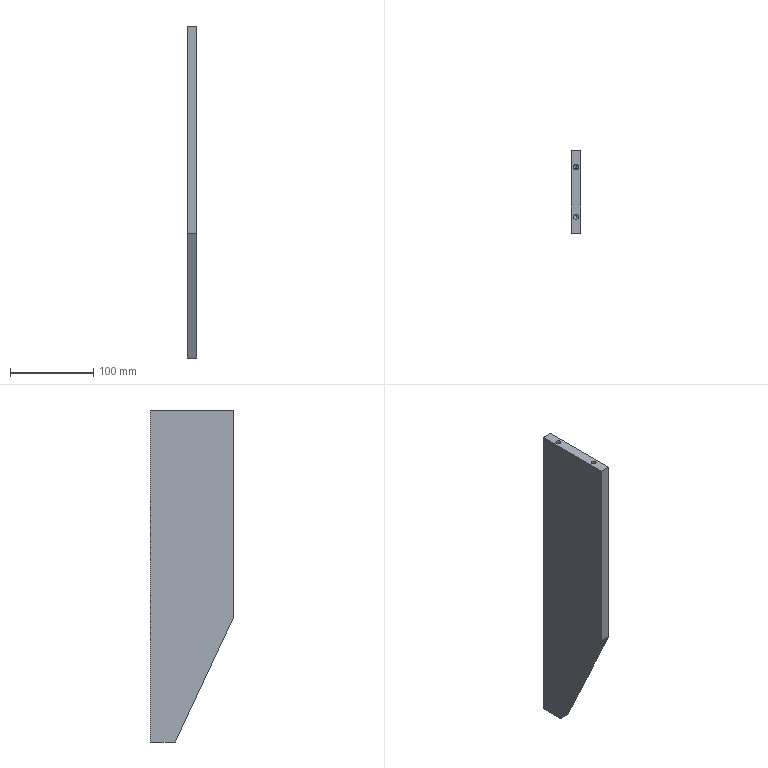Component | SolidWorks | 8TC-A15004-80-03A-1 | 1 solid | 31 faces | box 12 x 100 x 400 mm | volume 414014 mm3 | cylinder 12 | cone 12 | plane 7 | commonest cylinder face diameters 6 x12 | material A3
build123d program:
from build123d import *

# Parameters (mm, degrees)
BOSS_EXTRUDE1_DEPTH   = 6
M6_TAPPED_HOLE1_D     = 6
M6_TAPPED_HOLE1_DEPTH = 17
M6_TAPPED_HOLE1_TIP   = 1.803
M6_TAPPED_HOLE2_D     = 6
M6_TAPPED_HOLE2_DEPTH = 17
M6_TAPPED_HOLE2_TIP   = 1.803


with BuildPart() as part:
    # Sketch1 → Boss-Extrude1 (new, symmetric)
    with BuildSketch(Plane(origin=(0, 0, 0), x_dir=(1, 0, 0), z_dir=(0, 1, 0))):
        Polygon((0, 0), (0, 400), (30, 400), (100, 250), (100, 0), align=None)
    extrude(amount=BOSS_EXTRUDE1_DEPTH, both=True)

    # M6 Tapped Hole1
    with Locations(Plane.XY):
        with Locations((20, 0), (80, 0)):
            Hole(M6_TAPPED_HOLE1_D / 2, depth=M6_TAPPED_HOLE1_DEPTH)
            with Locations((0, 0, -(M6_TAPPED_HOLE1_DEPTH + M6_TAPPED_HOLE1_TIP / 2))):  # 118° drill point
                Cone(0, M6_TAPPED_HOLE1_D / 2, M6_TAPPED_HOLE1_TIP, mode=Mode.SUBTRACT)

    # M6 Tapped Hole2
    with Locations(Plane.ZY):
        with Locations((-50, 0), (-150, 0), (-250, 0), (-350, 0)):
            Hole(M6_TAPPED_HOLE2_D / 2, depth=M6_TAPPED_HOLE2_DEPTH)
            with Locations((0, 0, -(M6_TAPPED_HOLE2_DEPTH + M6_TAPPED_HOLE2_TIP / 2))):  # 118° drill point
                Cone(0, M6_TAPPED_HOLE2_D / 2, M6_TAPPED_HOLE2_TIP, mode=Mode.SUBTRACT)


solid = part.part

# Placed as in the assembly
solid = solid.moved(Location((54, -7.5, 0), (0, 0, -90)))
STEP:
#1=COLOUR_RGB('',0.7922,0.8196,0.9333);
#2=FILL_AREA_STYLE_COLOUR('',#1);
#3=FILL_AREA_STYLE('',(#2));
#4=SURFACE_STYLE_FILL_AREA(#3);
#5=SURFACE_SIDE_STYLE('',(#4));
#6=SURFACE_STYLE_USAGE(.BOTH.,#5);
#7=PRESENTATION_STYLE_ASSIGNMENT((#6));
#8=CARTESIAN_POINT('',(2.126,-0.9646,-2.087));
#9=VERTEX_POINT('',#8);
#10=CARTESIAN_POINT('',(2.126,-0.9646,-1.85));
#11=VERTEX_POINT('',#10);
#12=CARTESIAN_POINT('',(2.126,-0.9646,-1.969));
#13=DIRECTION('',(-0.,1.,0.));
#14=DIRECTION('',(0.,0.,1.));
#15=AXIS2_PLACEMENT_3D('',#12,#13,#14);
#16=CIRCLE('',#15,0.1181);
#17=EDGE_CURVE('',#9,#11,#16,.T.);
#18=ORIENTED_EDGE('',*,*,#17,.F.);
#19=CARTESIAN_POINT('',(2.126,-0.2953,-2.087));
#20=VERTEX_POINT('',#19);
#21=CARTESIAN_POINT('',(2.126,-0.2953,-2.087));
#22=DIRECTION('',(-0.,1.,0.));
#23=VECTOR('',#22,39.37);
#24=LINE('',#21,#23);
#25=EDGE_CURVE('',#9,#20,#24,.T.);
#26=ORIENTED_EDGE('',*,*,#25,.T.);
#27=CARTESIAN_POINT('',(2.126,-0.2953,-1.85));
#28=VERTEX_POINT('',#27);
#29=CARTESIAN_POINT('',(2.126,-0.2953,-1.969));
#30=DIRECTION('',(-0.,1.,0.));
#31=DIRECTION('',(0.,0.,1.));
#32=AXIS2_PLACEMENT_3D('',#29,#30,#31);
#33=CIRCLE('',#32,0.1181);
#34=EDGE_CURVE('',#20,#28,#33,.T.);
#35=ORIENTED_EDGE('',*,*,#34,.T.);
#36=CARTESIAN_POINT('',(2.126,-0.2953,-1.85));
#37=DIRECTION('',(-0.,1.,0.));
#38=VECTOR('',#37,39.37);
#39=LINE('',#36,#38);
#40=EDGE_CURVE('',#11,#28,#39,.T.);
#41=ORIENTED_EDGE('',*,*,#40,.F.);
#42=EDGE_LOOP('',(#18,#26,#35,#41));
#43=FACE_OUTER_BOUND('',#42,.T.);
#44=CARTESIAN_POINT('',(2.126,-0.2953,-1.969));
#45=DIRECTION('',(-0.,1.,0.));
#46=DIRECTION('',(0.,0.,1.));
#47=AXIS2_PLACEMENT_3D('',#44,#45,#46);
#48=CYLINDRICAL_SURFACE('',#47,0.1181);
#49=ADVANCED_FACE('',(#43),#48,.F.);
#50=CARTESIAN_POINT('',(2.126,-1.036,-1.969));
#51=VERTEX_POINT('',#50);
#52=CARTESIAN_POINT('',(2.126,-0.9646,-1.85));
#53=DIRECTION('',(-0.,0.515,0.8572));
#54=VECTOR('',#53,39.37);
#55=LINE('',#52,#54);
#56=EDGE_CURVE('',#51,#11,#55,.T.);
#57=ORIENTED_EDGE('',*,*,#56,.F.);
#58=CARTESIAN_POINT('',(2.126,-0.9646,-2.087));
#59=DIRECTION('',(0.,0.515,-0.8572));
#60=VECTOR('',#59,39.37);
#61=LINE('',#58,#60);
#62=EDGE_CURVE('',#51,#9,#61,.T.);
#63=ORIENTED_EDGE('',*,*,#62,.T.);
#64=ORIENTED_EDGE('',*,*,#17,.T.);
#65=EDGE_LOOP('',(#57,#63,#64));
#66=FACE_OUTER_BOUND('',#65,.T.);
#67=CARTESIAN_POINT('',(2.126,-0.9646,-1.969));
#68=DIRECTION('',(-0.,1.,0.));
#69=DIRECTION('',(0.,0.,1.));
#70=AXIS2_PLACEMENT_3D('',#67,#68,#69);
#71=CONICAL_SURFACE('',#70,0.1181,1.03);
#72=ADVANCED_FACE('',(#66),#71,.F.);
#73=CARTESIAN_POINT('',(2.126,-0.9646,-6.024));
#74=VERTEX_POINT('',#73);
#75=CARTESIAN_POINT('',(2.126,-0.9646,-5.787));
#76=VERTEX_POINT('',#75);
#77=CARTESIAN_POINT('',(2.126,-0.9646,-5.906));
#78=DIRECTION('',(-0.,1.,0.));
#79=DIRECTION('',(0.,0.,1.));
#80=AXIS2_PLACEMENT_3D('',#77,#78,#79);
#81=CIRCLE('',#80,0.1181);
#82=EDGE_CURVE('',#74,#76,#81,.T.);
#83=ORIENTED_EDGE('',*,*,#82,.F.);
#84=CARTESIAN_POINT('',(2.126,-0.2953,-6.024));
#85=VERTEX_POINT('',#84);
#86=CARTESIAN_POINT('',(2.126,-0.2953,-6.024));
#87=DIRECTION('',(-0.,1.,0.));
#88=VECTOR('',#87,39.37);
#89=LINE('',#86,#88);
#90=EDGE_CURVE('',#74,#85,#89,.T.);
#91=ORIENTED_EDGE('',*,*,#90,.T.);
#92=CARTESIAN_POINT('',(2.126,-0.2953,-5.787));
#93=VERTEX_POINT('',#92);
#94=CARTESIAN_POINT('',(2.126,-0.2953,-5.906));
#95=DIRECTION('',(-0.,1.,0.));
#96=DIRECTION('',(0.,0.,1.));
#97=AXIS2_PLACEMENT_3D('',#94,#95,#96);
#98=CIRCLE('',#97,0.1181);
#99=EDGE_CURVE('',#85,#93,#98,.T.);
#100=ORIENTED_EDGE('',*,*,#99,.T.);
#101=CARTESIAN_POINT('',(2.126,-0.2953,-5.787));
#102=DIRECTION('',(-0.,1.,0.));
#103=VECTOR('',#102,39.37);
#104=LINE('',#101,#103);
#105=EDGE_CURVE('',#76,#93,#104,.T.);
#106=ORIENTED_EDGE('',*,*,#105,.F.);
#107=EDGE_LOOP('',(#83,#91,#100,#106));
#108=FACE_OUTER_BOUND('',#107,.T.);
#109=CARTESIAN_POINT('',(2.126,-0.2953,-5.906));
#110=DIRECTION('',(-0.,1.,0.));
#111=DIRECTION('',(0.,0.,1.));
#112=AXIS2_PLACEMENT_3D('',#109,#110,#111);
#113=CYLINDRICAL_SURFACE('',#112,0.1181);
#114=ADVANCED_FACE('',(#108),#113,.F.);
#115=CARTESIAN_POINT('',(2.126,-1.036,-5.906));
#116=VERTEX_POINT('',#115);
#117=CARTESIAN_POINT('',(2.126,-0.9646,-5.787));
#118=DIRECTION('',(-0.,0.515,0.8572));
#119=VECTOR('',#118,39.37);
#120=LINE('',#117,#119);
#121=EDGE_CURVE('',#116,#76,#120,.T.);
#122=ORIENTED_EDGE('',*,*,#121,.F.);
#123=CARTESIAN_POINT('',(2.126,-0.9646,-6.024));
#124=DIRECTION('',(0.,0.515,-0.8572));
#125=VECTOR('',#124,39.37);
#126=LINE('',#123,#125);
#127=EDGE_CURVE('',#116,#74,#126,.T.);
#128=ORIENTED_EDGE('',*,*,#127,.T.);
#129=ORIENTED_EDGE('',*,*,#82,.T.);
#130=EDGE_LOOP('',(#122,#128,#129));
#131=FACE_OUTER_BOUND('',#130,.T.);
#132=CARTESIAN_POINT('',(2.126,-0.9646,-5.906));
#133=DIRECTION('',(-0.,1.,0.));
#134=DIRECTION('',(0.,0.,1.));
#135=AXIS2_PLACEMENT_3D('',#132,#133,#134);
#136=CONICAL_SURFACE('',#135,0.1181,1.03);
#137=ADVANCED_FACE('',(#131),#136,.F.);
#138=CARTESIAN_POINT('',(2.126,-0.9646,-9.961));
#139=VERTEX_POINT('',#138);
#140=CARTESIAN_POINT('',(2.126,-0.9646,-9.724));
#141=VERTEX_POINT('',#140);
#142=CARTESIAN_POINT('',(2.126,-0.9646,-9.843));
#143=DIRECTION('',(-0.,1.,0.));
#144=DIRECTION('',(0.,0.,1.));
#145=AXIS2_PLACEMENT_3D('',#142,#143,#144);
#146=CIRCLE('',#145,0.1181);
#147=EDGE_CURVE('',#139,#141,#146,.T.);
#148=ORIENTED_EDGE('',*,*,#147,.F.);
#149=CARTESIAN_POINT('',(2.126,-0.2953,-9.961));
#150=VERTEX_POINT('',#149);
#151=CARTESIAN_POINT('',(2.126,-0.2953,-9.961));
#152=DIRECTION('',(-0.,1.,0.));
#153=VECTOR('',#152,39.37);
#154=LINE('',#151,#153);
#155=EDGE_CURVE('',#139,#150,#154,.T.);
#156=ORIENTED_EDGE('',*,*,#155,.T.);
#157=CARTESIAN_POINT('',(2.126,-0.2953,-9.724));
#158=VERTEX_POINT('',#157);
#159=CARTESIAN_POINT('',(2.126,-0.2953,-9.843));
#160=DIRECTION('',(-0.,1.,0.));
#161=DIRECTION('',(0.,0.,1.));
#162=AXIS2_PLACEMENT_3D('',#159,#160,#161);
#163=CIRCLE('',#162,0.1181);
#164=EDGE_CURVE('',#150,#158,#163,.T.);
#165=ORIENTED_EDGE('',*,*,#164,.T.);
#166=CARTESIAN_POINT('',(2.126,-0.2953,-9.724));
#167=DIRECTION('',(-0.,1.,0.));
#168=VECTOR('',#167,39.37);
#169=LINE('',#166,#168);
#170=EDGE_CURVE('',#141,#158,#169,.T.);
#171=ORIENTED_EDGE('',*,*,#170,.F.);
#172=EDGE_LOOP('',(#148,#156,#165,#171));
#173=FACE_OUTER_BOUND('',#172,.T.);
#174=CARTESIAN_POINT('',(2.126,-0.2953,-9.843));
#175=DIRECTION('',(-0.,1.,0.));
#176=DIRECTION('',(0.,0.,1.));
#177=AXIS2_PLACEMENT_3D('',#174,#175,#176);
#178=CYLINDRICAL_SURFACE('',#177,0.1181);
#179=ADVANCED_FACE('',(#173),#178,.F.);
#180=CARTESIAN_POINT('',(2.126,-1.036,-9.843));
#181=VERTEX_POINT('',#180);
#182=CARTESIAN_POINT('',(2.126,-0.9646,-9.724));
#183=DIRECTION('',(-0.,0.515,0.8572));
#184=VECTOR('',#183,39.37);
#185=LINE('',#182,#184);
#186=EDGE_CURVE('',#181,#141,#185,.T.);
#187=ORIENTED_EDGE('',*,*,#186,.F.);
#188=CARTESIAN_POINT('',(2.126,-0.9646,-9.961));
#189=DIRECTION('',(0.,0.515,-0.8572));
#190=VECTOR('',#189,39.37);
#191=LINE('',#188,#190);
#192=EDGE_CURVE('',#181,#139,#191,.T.);
#193=ORIENTED_EDGE('',*,*,#192,.T.);
#194=ORIENTED_EDGE('',*,*,#147,.T.);
#195=EDGE_LOOP('',(#187,#193,#194));
#196=FACE_OUTER_BOUND('',#195,.T.);
#197=CARTESIAN_POINT('',(2.126,-0.9646,-9.843));
#198=DIRECTION('',(-0.,1.,0.));
#199=DIRECTION('',(0.,0.,1.));
#200=AXIS2_PLACEMENT_3D('',#197,#198,#199);
#201=CONICAL_SURFACE('',#200,0.1181,1.03);
#202=ADVANCED_FACE('',(#196),#201,.F.);
#203=CARTESIAN_POINT('',(2.126,-0.9646,-13.898));
#204=VERTEX_POINT('',#203);
#205=CARTESIAN_POINT('',(2.126,-0.9646,-13.661));
#206=VERTEX_POINT('',#205);
#207=CARTESIAN_POINT('',(2.126,-0.9646,-13.78));
#208=DIRECTION('',(-0.,1.,0.));
#209=DIRECTION('',(0.,0.,1.));
#210=AXIS2_PLACEMENT_3D('',#207,#208,#209);
#211=CIRCLE('',#210,0.1181);
#212=EDGE_CURVE('',#204,#206,#211,.T.);
#213=ORIENTED_EDGE('',*,*,#212,.F.);
#214=CARTESIAN_POINT('',(2.126,-0.2953,-13.898));
#215=VERTEX_POINT('',#214);
#216=CARTESIAN_POINT('',(2.126,-0.2953,-13.898));
#217=DIRECTION('',(-0.,1.,0.));
#218=VECTOR('',#217,39.37);
#219=LINE('',#216,#218);
#220=EDGE_CURVE('',#204,#215,#219,.T.);
#221=ORIENTED_EDGE('',*,*,#220,.T.);
#222=CARTESIAN_POINT('',(2.126,-0.2953,-13.661));
#223=VERTEX_POINT('',#222);
#224=CARTESIAN_POINT('',(2.126,-0.2953,-13.78));
#225=DIRECTION('',(-0.,1.,0.));
#226=DIRECTION('',(0.,0.,1.));
#227=AXIS2_PLACEMENT_3D('',#224,#225,#226);
#228=CIRCLE('',#227,0.1181);
#229=EDGE_CURVE('',#215,#223,#228,.T.);
#230=ORIENTED_EDGE('',*,*,#229,.T.);
#231=CARTESIAN_POINT('',(2.126,-0.2953,-13.661));
#232=DIRECTION('',(-0.,1.,0.));
#233=VECTOR('',#232,39.37);
#234=LINE('',#231,#233);
#235=EDGE_CURVE('',#206,#223,#234,.T.);
#236=ORIENTED_EDGE('',*,*,#235,.F.);
#237=EDGE_LOOP('',(#213,#221,#230,#236));
#238=FACE_OUTER_BOUND('',#237,.T.);
#239=CARTESIAN_POINT('',(2.126,-0.2953,-13.78));
#240=DIRECTION('',(-0.,1.,0.));
#241=DIRECTION('',(0.,0.,1.));
#242=AXIS2_PLACEMENT_3D('',#239,#240,#241);
#243=CYLINDRICAL_SURFACE('',#242,0.1181);
#244=ADVANCED_FACE('',(#238),#243,.F.);
#245=CARTESIAN_POINT('',(2.126,-1.036,-13.78));
#246=VERTEX_POINT('',#245);
#247=CARTESIAN_POINT('',(2.126,-0.9646,-13.661));
#248=DIRECTION('',(-0.,0.515,0.8572));
#249=VECTOR('',#248,39.37);
#250=LINE('',#247,#249);
#251=EDGE_CURVE('',#246,#206,#250,.T.);
#252=ORIENTED_EDGE('',*,*,#251,.F.);
#253=CARTESIAN_POINT('',(2.126,-0.9646,-13.898));
#254=DIRECTION('',(0.,0.515,-0.8572));
#255=VECTOR('',#254,39.37);
#256=LINE('',#253,#255);
#257=EDGE_CURVE('',#246,#204,#256,.T.);
#258=ORIENTED_EDGE('',*,*,#257,.T.);
#259=ORIENTED_EDGE('',*,*,#212,.T.);
#260=EDGE_LOOP('',(#252,#258,#259));
#261=FACE_OUTER_BOUND('',#260,.T.);
#262=CARTESIAN_POINT('',(2.126,-0.9646,-13.78));
#263=DIRECTION('',(-0.,1.,0.));
#264=DIRECTION('',(0.,0.,1.));
#265=AXIS2_PLACEMENT_3D('',#262,#263,#264);
#266=CONICAL_SURFACE('',#265,0.1181,1.03);
#267=ADVANCED_FACE('',(#261),#266,.F.);
#268=CARTESIAN_POINT('',(2.126,-0.9646,-0.6693));
#269=VERTEX_POINT('',#268);
#270=CARTESIAN_POINT('',(2.126,-1.201,-0.6693));
#271=VERTEX_POINT('',#270);
#272=CARTESIAN_POINT('',(2.126,-1.083,-0.6693));
#273=DIRECTION('',(-0.,-0.,1.));
#274=DIRECTION('',(0.,-1.,0.));
#275=AXIS2_PLACEMENT_3D('',#272,#273,#274);
#276=CIRCLE('',#275,0.1181);
#277=EDGE_CURVE('',#269,#271,#276,.T.);
#278=ORIENTED_EDGE('',*,*,#277,.F.);
#279=CARTESIAN_POINT('',(2.126,-0.9646,-0.));
#280=VERTEX_POINT('',#279);
#281=CARTESIAN_POINT('',(2.126,-0.9646,-0.));
#282=DIRECTION('',(-0.,-0.,1.));
#283=VECTOR('',#282,39.37);
#284=LINE('',#281,#283);
#285=EDGE_CURVE('',#269,#280,#284,.T.);
#286=ORIENTED_EDGE('',*,*,#285,.T.);
#287=CARTESIAN_POINT('',(2.126,-1.201,-0.));
#288=VERTEX_POINT('',#287);
#289=CARTESIAN_POINT('',(2.126,-1.083,-0.));
#290=DIRECTION('',(-0.,-0.,1.));
#291=DIRECTION('',(0.,-1.,0.));
#292=AXIS2_PLACEMENT_3D('',#289,#290,#291);
#293=CIRCLE('',#292,0.1181);
#294=EDGE_CURVE('',#280,#288,#293,.T.);
#295=ORIENTED_EDGE('',*,*,#294,.T.);
#296=CARTESIAN_POINT('',(2.126,-1.201,-0.));
#297=DIRECTION('',(-0.,-0.,1.));
#298=VECTOR('',#297,39.37);
#299=LINE('',#296,#298);
#300=EDGE_CURVE('',#271,#288,#299,.T.);
#301=ORIENTED_EDGE('',*,*,#300,.F.);
#302=EDGE_LOOP('',(#278,#286,#295,#301));
#303=FACE_OUTER_BOUND('',#302,.T.);
#304=CARTESIAN_POINT('',(2.126,-1.083,-0.));
#305=DIRECTION('',(-0.,-0.,1.));
#306=DIRECTION('',(0.,-1.,0.));
#307=AXIS2_PLACEMENT_3D('',#304,#305,#306);
#308=CYLINDRICAL_SURFACE('',#307,0.1181);
#309=ADVANCED_FACE('',(#303),#308,.F.);
#310=CARTESIAN_POINT('',(2.126,-1.083,-0.7403));
#311=VERTEX_POINT('',#310);
#312=CARTESIAN_POINT('',(2.126,-1.201,-0.6693));
#313=DIRECTION('',(0.,-0.8572,0.515));
#314=VECTOR('',#313,39.37);
#315=LINE('',#312,#314);
#316=EDGE_CURVE('',#311,#271,#315,.T.);
#317=ORIENTED_EDGE('',*,*,#316,.F.);
#318=CARTESIAN_POINT('',(2.126,-0.9646,-0.6693));
#319=DIRECTION('',(-0.,0.8572,0.515));
#320=VECTOR('',#319,39.37);
#321=LINE('',#318,#320);
#322=EDGE_CURVE('',#311,#269,#321,.T.);
#323=ORIENTED_EDGE('',*,*,#322,.T.);
#324=ORIENTED_EDGE('',*,*,#277,.T.);
#325=EDGE_LOOP('',(#317,#323,#324));
#326=FACE_OUTER_BOUND('',#325,.T.);
#327=CARTESIAN_POINT('',(2.126,-1.083,-0.6693));
#328=DIRECTION('',(-0.,-0.,1.));
#329=DIRECTION('',(0.,-1.,0.));
#330=AXIS2_PLACEMENT_3D('',#327,#328,#329);
#331=CONICAL_SURFACE('',#330,0.1181,1.03);
#332=ADVANCED_FACE('',(#326),#331,.F.);
#333=CARTESIAN_POINT('',(2.126,-3.327,-0.6693));
#334=VERTEX_POINT('',#333);
#335=CARTESIAN_POINT('',(2.126,-3.563,-0.6693));
#336=VERTEX_POINT('',#335);
#337=CARTESIAN_POINT('',(2.126,-3.445,-0.6693));
#338=DIRECTION('',(-0.,-0.,1.));
#339=DIRECTION('',(0.,-1.,0.));
#340=AXIS2_PLACEMENT_3D('',#337,#338,#339);
#341=CIRCLE('',#340,0.1181);
#342=EDGE_CURVE('',#334,#336,#341,.T.);
#343=ORIENTED_EDGE('',*,*,#342,.F.);
#344=CARTESIAN_POINT('',(2.126,-3.327,-0.));
#345=VERTEX_POINT('',#344);
#346=CARTESIAN_POINT('',(2.126,-3.327,-0.));
#347=DIRECTION('',(-0.,-0.,1.));
#348=VECTOR('',#347,39.37);
#349=LINE('',#346,#348);
#350=EDGE_CURVE('',#334,#345,#349,.T.);
#351=ORIENTED_EDGE('',*,*,#350,.T.);
#352=CARTESIAN_POINT('',(2.126,-3.563,-0.));
#353=VERTEX_POINT('',#352);
#354=CARTESIAN_POINT('',(2.126,-3.445,-0.));
#355=DIRECTION('',(-0.,-0.,1.));
#356=DIRECTION('',(0.,-1.,0.));
#357=AXIS2_PLACEMENT_3D('',#354,#355,#356);
#358=CIRCLE('',#357,0.1181);
#359=EDGE_CURVE('',#345,#353,#358,.T.);
#360=ORIENTED_EDGE('',*,*,#359,.T.);
#361=CARTESIAN_POINT('',(2.126,-3.563,-0.));
#362=DIRECTION('',(-0.,-0.,1.));
#363=VECTOR('',#362,39.37);
#364=LINE('',#361,#363);
#365=EDGE_CURVE('',#336,#353,#364,.T.);
#366=ORIENTED_EDGE('',*,*,#365,.F.);
#367=EDGE_LOOP('',(#343,#351,#360,#366));
#368=FACE_OUTER_BOUND('',#367,.T.);
#369=CARTESIAN_POINT('',(2.126,-3.445,-0.));
#370=DIRECTION('',(-0.,-0.,1.));
#371=DIRECTION('',(0.,-1.,0.));
#372=AXIS2_PLACEMENT_3D('',#369,#370,#371);
#373=CYLINDRICAL_SURFACE('',#372,0.1181);
#374=ADVANCED_FACE('',(#368),#373,.F.);
#375=CARTESIAN_POINT('',(2.126,-3.445,-0.7403));
#376=VERTEX_POINT('',#375);
#377=CARTESIAN_POINT('',(2.126,-3.563,-0.6693));
#378=DIRECTION('',(0.,-0.8572,0.515));
#379=VECTOR('',#378,39.37);
#380=LINE('',#377,#379);
#381=EDGE_CURVE('',#376,#336,#380,.T.);
#382=ORIENTED_EDGE('',*,*,#381,.F.);
#383=CARTESIAN_POINT('',(2.126,-3.327,-0.6693));
#384=DIRECTION('',(-0.,0.8572,0.515));
#385=VECTOR('',#384,39.37);
#386=LINE('',#383,#385);
#387=EDGE_CURVE('',#376,#334,#386,.T.);
#388=ORIENTED_EDGE('',*,*,#387,.T.);
#389=ORIENTED_EDGE('',*,*,#342,.T.);
#390=EDGE_LOOP('',(#382,#388,#389));
#391=FACE_OUTER_BOUND('',#390,.T.);
#392=CARTESIAN_POINT('',(2.126,-3.445,-0.6693));
#393=DIRECTION('',(-0.,-0.,1.));
#394=DIRECTION('',(0.,-1.,0.));
#395=AXIS2_PLACEMENT_3D('',#392,#393,#394);
#396=CONICAL_SURFACE('',#395,0.1181,1.03);
#397=ADVANCED_FACE('',(#391),#396,.F.);
#398=CARTESIAN_POINT('',(2.126,-1.083,-0.));
#399=DIRECTION('',(-0.,-0.,1.));
#400=DIRECTION('',(0.,-1.,0.));
#401=AXIS2_PLACEMENT_3D('',#398,#399,#400);
#402=CIRCLE('',#401,0.1181);
#403=EDGE_CURVE('',#288,#280,#402,.T.);
#404=ORIENTED_EDGE('',*,*,#403,.F.);
#405=ORIENTED_EDGE('',*,*,#294,.F.);
#406=EDGE_LOOP('',(#404,#405));
#407=FACE_BOUND('',#406,.T.);
#408=CARTESIAN_POINT('',(2.126,-3.445,-0.));
#409=DIRECTION('',(-0.,-0.,1.));
#410=DIRECTION('',(0.,-1.,0.));
#411=AXIS2_PLACEMENT_3D('',#408,#409,#410);
#412=CIRCLE('',#411,0.1181);
#413=EDGE_CURVE('',#353,#345,#412,.T.);
#414=ORIENTED_EDGE('',*,*,#413,.F.);
#415=ORIENTED_EDGE('',*,*,#359,.F.);
#416=EDGE_LOOP('',(#414,#415));
#417=FACE_BOUND('',#416,.T.);
#418=CARTESIAN_POINT('',(1.89,-0.2953,-0.));
#419=VERTEX_POINT('',#418);
#420=CARTESIAN_POINT('',(1.89,-4.232,-0.));
#421=VERTEX_POINT('',#420);
#422=CARTESIAN_POINT('',(1.89,-4.232,-0.));
#423=DIRECTION('',(0.,-1.,0.));
#424=VECTOR('',#423,39.37);
#425=LINE('',#422,#424);
#426=EDGE_CURVE('',#419,#421,#425,.T.);
#427=ORIENTED_EDGE('',*,*,#426,.T.);
#428=CARTESIAN_POINT('',(2.362,-4.232,-0.));
#429=VERTEX_POINT('',#428);
#430=CARTESIAN_POINT('',(2.362,-4.232,-0.));
#431=DIRECTION('',(-1.,-0.,-0.));
#432=VECTOR('',#431,39.37);
#433=LINE('',#430,#432);
#434=EDGE_CURVE('',#429,#421,#433,.T.);
#435=ORIENTED_EDGE('',*,*,#434,.F.);
#436=CARTESIAN_POINT('',(2.362,-0.2953,-0.));
#437=VERTEX_POINT('',#436);
#438=CARTESIAN_POINT('',(2.362,-4.232,-0.));
#439=DIRECTION('',(0.,-1.,0.));
#440=VECTOR('',#439,39.37);
#441=LINE('',#438,#440);
#442=EDGE_CURVE('',#437,#429,#441,.T.);
#443=ORIENTED_EDGE('',*,*,#442,.F.);
#444=CARTESIAN_POINT('',(2.362,-0.2953,-0.));
#445=DIRECTION('',(-1.,-0.,-0.));
#446=VECTOR('',#445,39.37);
#447=LINE('',#444,#446);
#448=EDGE_CURVE('',#437,#419,#447,.T.);
#449=ORIENTED_EDGE('',*,*,#448,.T.);
#450=EDGE_LOOP('',(#427,#435,#443,#449));
#451=FACE_OUTER_BOUND('',#450,.T.);
#452=CARTESIAN_POINT('',(2.362,-4.232,-0.));
#453=DIRECTION('',(0.,0.,-1.));
#454=DIRECTION('',(-0.,1.,0.));
#455=AXIS2_PLACEMENT_3D('',#452,#453,#454);
#456=PLANE('',#455);
#457=ADVANCED_FACE('',(#407,#417,#451),#456,.F.);
#458=CARTESIAN_POINT('',(1.89,-4.232,-9.843));
#459=VERTEX_POINT('',#458);
#460=CARTESIAN_POINT('',(1.89,-4.232,-9.843));
#461=DIRECTION('',(0.,0.,-1.));
#462=VECTOR('',#461,39.37);
#463=LINE('',#460,#462);
#464=EDGE_CURVE('',#421,#459,#463,.T.);
#465=ORIENTED_EDGE('',*,*,#464,.T.);
#466=CARTESIAN_POINT('',(2.362,-4.232,-9.843));
#467=VERTEX_POINT('',#466);
#468=CARTESIAN_POINT('',(2.362,-4.232,-9.843));
#469=DIRECTION('',(-1.,-0.,-0.));
#470=VECTOR('',#469,39.37);
#471=LINE('',#468,#470);
#472=EDGE_CURVE('',#467,#459,#471,.T.);
#473=ORIENTED_EDGE('',*,*,#472,.F.);
#474=CARTESIAN_POINT('',(2.362,-4.232,-9.843));
#475=DIRECTION('',(0.,0.,-1.));
#476=VECTOR('',#475,39.37);
#477=LINE('',#474,#476);
#478=EDGE_CURVE('',#429,#467,#477,.T.);
#479=ORIENTED_EDGE('',*,*,#478,.F.);
#480=ORIENTED_EDGE('',*,*,#434,.T.);
#481=EDGE_LOOP('',(#465,#473,#479,#480));
#482=FACE_OUTER_BOUND('',#481,.T.);
#483=CARTESIAN_POINT('',(2.362,-4.232,-9.843));
#484=DIRECTION('',(-0.,1.,0.));
#485=DIRECTION('',(-0.,-0.,1.));
#486=AXIS2_PLACEMENT_3D('',#483,#484,#485);
#487=PLANE('',#486);
#488=ADVANCED_FACE('',(#482),#487,.F.);
#489=CARTESIAN_POINT('',(1.89,-1.476,-15.748));
#490=VERTEX_POINT('',#489);
#491=CARTESIAN_POINT('',(1.89,-1.476,-15.748));
#492=DIRECTION('',(-0.,0.4229,-0.9062));
#493=VECTOR('',#492,39.37);
#494=LINE('',#491,#493);
#495=EDGE_CURVE('',#459,#490,#494,.T.);
#496=ORIENTED_EDGE('',*,*,#495,.T.);
#497=CARTESIAN_POINT('',(2.362,-1.476,-15.748));
#498=VERTEX_POINT('',#497);
#499=CARTESIAN_POINT('',(2.362,-1.476,-15.748));
#500=DIRECTION('',(-1.,-0.,-0.));
#501=VECTOR('',#500,39.37);
#502=LINE('',#499,#501);
#503=EDGE_CURVE('',#498,#490,#502,.T.);
#504=ORIENTED_EDGE('',*,*,#503,.F.);
#505=CARTESIAN_POINT('',(2.362,-1.476,-15.748));
#506=DIRECTION('',(-0.,0.4229,-0.9062));
#507=VECTOR('',#506,39.37);
#508=LINE('',#505,#507);
#509=EDGE_CURVE('',#467,#498,#508,.T.);
#510=ORIENTED_EDGE('',*,*,#509,.F.);
#511=ORIENTED_EDGE('',*,*,#472,.T.);
#512=EDGE_LOOP('',(#496,#504,#510,#511));
#513=FACE_OUTER_BOUND('',#512,.T.);
#514=CARTESIAN_POINT('',(2.362,-1.476,-15.748));
#515=DIRECTION('',(-0.,0.9062,0.4229));
#516=DIRECTION('',(0.,-0.4229,0.9062));
#517=AXIS2_PLACEMENT_3D('',#514,#515,#516);
#518=PLANE('',#517);
#519=ADVANCED_FACE('',(#513),#518,.F.);
#520=CARTESIAN_POINT('',(1.89,-0.2953,-15.748));
#521=VERTEX_POINT('',#520);
#522=CARTESIAN_POINT('',(1.89,-0.2953,-15.748));
#523=DIRECTION('',(-0.,1.,0.));
#524=VECTOR('',#523,39.37);
#525=LINE('',#522,#524);
#526=EDGE_CURVE('',#490,#521,#525,.T.);
#527=ORIENTED_EDGE('',*,*,#526,.T.);
#528=CARTESIAN_POINT('',(2.362,-0.2953,-15.748));
#529=VERTEX_POINT('',#528);
#530=CARTESIAN_POINT('',(2.362,-0.2953,-15.748));
#531=DIRECTION('',(-1.,-0.,-0.));
#532=VECTOR('',#531,39.37);
#533=LINE('',#530,#532);
#534=EDGE_CURVE('',#529,#521,#533,.T.);
#535=ORIENTED_EDGE('',*,*,#534,.F.);
#536=CARTESIAN_POINT('',(2.362,-0.2953,-15.748));
#537=DIRECTION('',(-0.,1.,0.));
#538=VECTOR('',#537,39.37);
#539=LINE('',#536,#538);
#540=EDGE_CURVE('',#498,#529,#539,.T.);
#541=ORIENTED_EDGE('',*,*,#540,.F.);
#542=ORIENTED_EDGE('',*,*,#503,.T.);
#543=EDGE_LOOP('',(#527,#535,#541,#542));
#544=FACE_OUTER_BOUND('',#543,.T.);
#545=CARTESIAN_POINT('',(2.362,-0.2953,-15.748));
#546=DIRECTION('',(-0.,-0.,1.));
#547=DIRECTION('',(0.,-1.,0.));
#548=AXIS2_PLACEMENT_3D('',#545,#546,#547);
#549=PLANE('',#548);
#550=ADVANCED_FACE('',(#544),#549,.F.);
#551=CARTESIAN_POINT('',(2.126,-0.2953,-1.969));
#552=DIRECTION('',(-0.,1.,0.));
#553=DIRECTION('',(0.,0.,1.));
#554=AXIS2_PLACEMENT_3D('',#551,#552,#553);
#555=CIRCLE('',#554,0.1181);
#556=EDGE_CURVE('',#28,#20,#555,.T.);
#557=ORIENTED_EDGE('',*,*,#556,.F.);
#558=ORIENTED_EDGE('',*,*,#34,.F.);
#559=EDGE_LOOP('',(#557,#558));
#560=FACE_BOUND('',#559,.T.);
#561=CARTESIAN_POINT('',(2.126,-0.2953,-5.906));
#562=DIRECTION('',(-0.,1.,0.));
#563=DIRECTION('',(0.,0.,1.));
#564=AXIS2_PLACEMENT_3D('',#561,#562,#563);
#565=CIRCLE('',#564,0.1181);
#566=EDGE_CURVE('',#93,#85,#565,.T.);
#567=ORIENTED_EDGE('',*,*,#566,.F.);
#568=ORIENTED_EDGE('',*,*,#99,.F.);
#569=EDGE_LOOP('',(#567,#568));
#570=FACE_BOUND('',#569,.T.);
#571=CARTESIAN_POINT('',(2.126,-0.2953,-9.843));
#572=DIRECTION('',(-0.,1.,0.));
#573=DIRECTION('',(0.,0.,1.));
#574=AXIS2_PLACEMENT_3D('',#571,#572,#573);
#575=CIRCLE('',#574,0.1181);
#576=EDGE_CURVE('',#158,#150,#575,.T.);
#577=ORIENTED_EDGE('',*,*,#576,.F.);
#578=ORIENTED_EDGE('',*,*,#164,.F.);
#579=EDGE_LOOP('',(#577,#578));
#580=FACE_BOUND('',#579,.T.);
#581=CARTESIAN_POINT('',(2.126,-0.2953,-13.78));
#582=DIRECTION('',(-0.,1.,0.));
#583=DIRECTION('',(0.,0.,1.));
#584=AXIS2_PLACEMENT_3D('',#581,#582,#583);
#585=CIRCLE('',#584,0.1181);
#586=EDGE_CURVE('',#223,#215,#585,.T.);
#587=ORIENTED_EDGE('',*,*,#586,.F.);
#588=ORIENTED_EDGE('',*,*,#229,.F.);
#589=EDGE_LOOP('',(#587,#588));
#590=FACE_BOUND('',#589,.T.);
#591=CARTESIAN_POINT('',(1.89,-0.2953,-0.));
#592=DIRECTION('',(-0.,-0.,1.));
#593=VECTOR('',#592,39.37);
#594=LINE('',#591,#593);
#595=EDGE_CURVE('',#521,#419,#594,.T.);
#596=ORIENTED_EDGE('',*,*,#595,.T.);
#597=ORIENTED_EDGE('',*,*,#448,.F.);
#598=CARTESIAN_POINT('',(2.362,-0.2953,-0.));
#599=DIRECTION('',(-0.,-0.,1.));
#600=VECTOR('',#599,39.37);
#601=LINE('',#598,#600);
#602=EDGE_CURVE('',#529,#437,#601,.T.);
#603=ORIENTED_EDGE('',*,*,#602,.F.);
#604=ORIENTED_EDGE('',*,*,#534,.T.);
#605=EDGE_LOOP('',(#596,#597,#603,#604));
#606=FACE_OUTER_BOUND('',#605,.T.);
#607=CARTESIAN_POINT('',(2.362,-0.2953,-0.));
#608=DIRECTION('',(0.,-1.,0.));
#609=DIRECTION('',(0.,0.,-1.));
#610=AXIS2_PLACEMENT_3D('',#607,#608,#609);
#611=PLANE('',#610);
#612=ADVANCED_FACE('',(#560,#570,#580,#590,#606),#611,.F.);
#613=ORIENTED_EDGE('',*,*,#442,.T.);
#614=ORIENTED_EDGE('',*,*,#478,.T.);
#615=ORIENTED_EDGE('',*,*,#509,.T.);
#616=ORIENTED_EDGE('',*,*,#540,.T.);
#617=ORIENTED_EDGE('',*,*,#602,.T.);
#618=EDGE_LOOP('',(#613,#614,#615,#616,#617));
#619=FACE_OUTER_BOUND('',#618,.T.);
#620=CARTESIAN_POINT('',(2.362,-0.2953,-0.));
#621=DIRECTION('',(-1.,-0.,-0.));
#622=DIRECTION('',(0.,0.,-1.));
#623=AXIS2_PLACEMENT_3D('',#620,#621,#622);
#624=PLANE('',#623);
#625=ADVANCED_FACE('',(#619),#624,.F.);
#626=ORIENTED_EDGE('',*,*,#426,.F.);
#627=ORIENTED_EDGE('',*,*,#595,.F.);
#628=ORIENTED_EDGE('',*,*,#526,.F.);
#629=ORIENTED_EDGE('',*,*,#495,.F.);
#630=ORIENTED_EDGE('',*,*,#464,.F.);
#631=EDGE_LOOP('',(#626,#627,#628,#629,#630));
#632=FACE_OUTER_BOUND('',#631,.T.);
#633=CARTESIAN_POINT('',(1.89,-0.2953,-0.));
#634=DIRECTION('',(-1.,-0.,-0.));
#635=DIRECTION('',(0.,0.,-1.));
#636=AXIS2_PLACEMENT_3D('',#633,#634,#635);
#637=PLANE('',#636);
#638=ADVANCED_FACE('',(#632),#637,.T.);
#639=ORIENTED_EDGE('',*,*,#387,.F.);
#640=ORIENTED_EDGE('',*,*,#381,.T.);
#641=CARTESIAN_POINT('',(2.126,-3.445,-0.6693));
#642=DIRECTION('',(-0.,-0.,1.));
#643=DIRECTION('',(0.,-1.,0.));
#644=AXIS2_PLACEMENT_3D('',#641,#642,#643);
#645=CIRCLE('',#644,0.1181);
#646=EDGE_CURVE('',#336,#334,#645,.T.);
#647=ORIENTED_EDGE('',*,*,#646,.T.);
#648=EDGE_LOOP('',(#639,#640,#647));
#649=FACE_OUTER_BOUND('',#648,.T.);
#650=CARTESIAN_POINT('',(2.126,-3.445,-0.6693));
#651=DIRECTION('',(-0.,-0.,1.));
#652=DIRECTION('',(0.,-1.,0.));
#653=AXIS2_PLACEMENT_3D('',#650,#651,#652);
#654=CONICAL_SURFACE('',#653,0.1181,1.03);
#655=ADVANCED_FACE('',(#649),#654,.F.);
#656=ORIENTED_EDGE('',*,*,#350,.F.);
#657=ORIENTED_EDGE('',*,*,#646,.F.);
#658=ORIENTED_EDGE('',*,*,#365,.T.);
#659=ORIENTED_EDGE('',*,*,#413,.T.);
#660=EDGE_LOOP('',(#656,#657,#658,#659));
#661=FACE_OUTER_BOUND('',#660,.T.);
#662=CARTESIAN_POINT('',(2.126,-3.445,-0.));
#663=DIRECTION('',(-0.,-0.,1.));
#664=DIRECTION('',(0.,-1.,0.));
#665=AXIS2_PLACEMENT_3D('',#662,#663,#664);
#666=CYLINDRICAL_SURFACE('',#665,0.1181);
#667=ADVANCED_FACE('',(#661),#666,.F.);
#668=ORIENTED_EDGE('',*,*,#322,.F.);
#669=ORIENTED_EDGE('',*,*,#316,.T.);
#670=CARTESIAN_POINT('',(2.126,-1.083,-0.6693));
#671=DIRECTION('',(-0.,-0.,1.));
#672=DIRECTION('',(0.,-1.,0.));
#673=AXIS2_PLACEMENT_3D('',#670,#671,#672);
#674=CIRCLE('',#673,0.1181);
#675=EDGE_CURVE('',#271,#269,#674,.T.);
#676=ORIENTED_EDGE('',*,*,#675,.T.);
#677=EDGE_LOOP('',(#668,#669,#676));
#678=FACE_OUTER_BOUND('',#677,.T.);
#679=CARTESIAN_POINT('',(2.126,-1.083,-0.6693));
#680=DIRECTION('',(-0.,-0.,1.));
#681=DIRECTION('',(0.,-1.,0.));
#682=AXIS2_PLACEMENT_3D('',#679,#680,#681);
#683=CONICAL_SURFACE('',#682,0.1181,1.03);
#684=ADVANCED_FACE('',(#678),#683,.F.);
#685=ORIENTED_EDGE('',*,*,#285,.F.);
#686=ORIENTED_EDGE('',*,*,#675,.F.);
#687=ORIENTED_EDGE('',*,*,#300,.T.);
#688=ORIENTED_EDGE('',*,*,#403,.T.);
#689=EDGE_LOOP('',(#685,#686,#687,#688));
#690=FACE_OUTER_BOUND('',#689,.T.);
#691=CARTESIAN_POINT('',(2.126,-1.083,-0.));
#692=DIRECTION('',(-0.,-0.,1.));
#693=DIRECTION('',(0.,-1.,0.));
#694=AXIS2_PLACEMENT_3D('',#691,#692,#693);
#695=CYLINDRICAL_SURFACE('',#694,0.1181);
#696=ADVANCED_FACE('',(#690),#695,.F.);
#697=ORIENTED_EDGE('',*,*,#257,.F.);
#698=ORIENTED_EDGE('',*,*,#251,.T.);
#699=CARTESIAN_POINT('',(2.126,-0.9646,-13.78));
#700=DIRECTION('',(-0.,1.,0.));
#701=DIRECTION('',(0.,0.,1.));
#702=AXIS2_PLACEMENT_3D('',#699,#700,#701);
#703=CIRCLE('',#702,0.1181);
#704=EDGE_CURVE('',#206,#204,#703,.T.);
#705=ORIENTED_EDGE('',*,*,#704,.T.);
#706=EDGE_LOOP('',(#697,#698,#705));
#707=FACE_OUTER_BOUND('',#706,.T.);
#708=CARTESIAN_POINT('',(2.126,-0.9646,-13.78));
#709=DIRECTION('',(-0.,1.,0.));
#710=DIRECTION('',(0.,0.,1.));
#711=AXIS2_PLACEMENT_3D('',#708,#709,#710);
#712=CONICAL_SURFACE('',#711,0.1181,1.03);
#713=ADVANCED_FACE('',(#707),#712,.F.);
#714=ORIENTED_EDGE('',*,*,#220,.F.);
#715=ORIENTED_EDGE('',*,*,#704,.F.);
#716=ORIENTED_EDGE('',*,*,#235,.T.);
#717=ORIENTED_EDGE('',*,*,#586,.T.);
#718=EDGE_LOOP('',(#714,#715,#716,#717));
#719=FACE_OUTER_BOUND('',#718,.T.);
#720=CARTESIAN_POINT('',(2.126,-0.2953,-13.78));
#721=DIRECTION('',(-0.,1.,0.));
#722=DIRECTION('',(0.,0.,1.));
#723=AXIS2_PLACEMENT_3D('',#720,#721,#722);
#724=CYLINDRICAL_SURFACE('',#723,0.1181);
#725=ADVANCED_FACE('',(#719),#724,.F.);
#726=ORIENTED_EDGE('',*,*,#192,.F.);
#727=ORIENTED_EDGE('',*,*,#186,.T.);
#728=CARTESIAN_POINT('',(2.126,-0.9646,-9.843));
#729=DIRECTION('',(-0.,1.,0.));
#730=DIRECTION('',(0.,0.,1.));
#731=AXIS2_PLACEMENT_3D('',#728,#729,#730);
#732=CIRCLE('',#731,0.1181);
#733=EDGE_CURVE('',#141,#139,#732,.T.);
#734=ORIENTED_EDGE('',*,*,#733,.T.);
#735=EDGE_LOOP('',(#726,#727,#734));
#736=FACE_OUTER_BOUND('',#735,.T.);
#737=CARTESIAN_POINT('',(2.126,-0.9646,-9.843));
#738=DIRECTION('',(-0.,1.,0.));
#739=DIRECTION('',(0.,0.,1.));
#740=AXIS2_PLACEMENT_3D('',#737,#738,#739);
#741=CONICAL_SURFACE('',#740,0.1181,1.03);
#742=ADVANCED_FACE('',(#736),#741,.F.);
#743=ORIENTED_EDGE('',*,*,#155,.F.);
#744=ORIENTED_EDGE('',*,*,#733,.F.);
#745=ORIENTED_EDGE('',*,*,#170,.T.);
#746=ORIENTED_EDGE('',*,*,#576,.T.);
#747=EDGE_LOOP('',(#743,#744,#745,#746));
#748=FACE_OUTER_BOUND('',#747,.T.);
#749=CARTESIAN_POINT('',(2.126,-0.2953,-9.843));
#750=DIRECTION('',(-0.,1.,0.));
#751=DIRECTION('',(0.,0.,1.));
#752=AXIS2_PLACEMENT_3D('',#749,#750,#751);
#753=CYLINDRICAL_SURFACE('',#752,0.1181);
#754=ADVANCED_FACE('',(#748),#753,.F.);
#755=ORIENTED_EDGE('',*,*,#127,.F.);
#756=ORIENTED_EDGE('',*,*,#121,.T.);
#757=CARTESIAN_POINT('',(2.126,-0.9646,-5.906));
#758=DIRECTION('',(-0.,1.,0.));
#759=DIRECTION('',(0.,0.,1.));
#760=AXIS2_PLACEMENT_3D('',#757,#758,#759);
#761=CIRCLE('',#760,0.1181);
#762=EDGE_CURVE('',#76,#74,#761,.T.);
#763=ORIENTED_EDGE('',*,*,#762,.T.);
#764=EDGE_LOOP('',(#755,#756,#763));
#765=FACE_OUTER_BOUND('',#764,.T.);
#766=CARTESIAN_POINT('',(2.126,-0.9646,-5.906));
#767=DIRECTION('',(-0.,1.,0.));
#768=DIRECTION('',(0.,0.,1.));
#769=AXIS2_PLACEMENT_3D('',#766,#767,#768);
#770=CONICAL_SURFACE('',#769,0.1181,1.03);
#771=ADVANCED_FACE('',(#765),#770,.F.);
#772=ORIENTED_EDGE('',*,*,#90,.F.);
#773=ORIENTED_EDGE('',*,*,#762,.F.);
#774=ORIENTED_EDGE('',*,*,#105,.T.);
#775=ORIENTED_EDGE('',*,*,#566,.T.);
#776=EDGE_LOOP('',(#772,#773,#774,#775));
#777=FACE_OUTER_BOUND('',#776,.T.);
#778=CARTESIAN_POINT('',(2.126,-0.2953,-5.906));
#779=DIRECTION('',(-0.,1.,0.));
#780=DIRECTION('',(0.,0.,1.));
#781=AXIS2_PLACEMENT_3D('',#778,#779,#780);
#782=CYLINDRICAL_SURFACE('',#781,0.1181);
#783=ADVANCED_FACE('',(#777),#782,.F.);
#784=ORIENTED_EDGE('',*,*,#62,.F.);
#785=ORIENTED_EDGE('',*,*,#56,.T.);
#786=CARTESIAN_POINT('',(2.126,-0.9646,-1.969));
#787=DIRECTION('',(-0.,1.,0.));
#788=DIRECTION('',(0.,0.,1.));
#789=AXIS2_PLACEMENT_3D('',#786,#787,#788);
#790=CIRCLE('',#789,0.1181);
#791=EDGE_CURVE('',#11,#9,#790,.T.);
#792=ORIENTED_EDGE('',*,*,#791,.T.);
#793=EDGE_LOOP('',(#784,#785,#792));
#794=FACE_OUTER_BOUND('',#793,.T.);
#795=CARTESIAN_POINT('',(2.126,-0.9646,-1.969));
#796=DIRECTION('',(-0.,1.,0.));
#797=DIRECTION('',(0.,0.,1.));
#798=AXIS2_PLACEMENT_3D('',#795,#796,#797);
#799=CONICAL_SURFACE('',#798,0.1181,1.03);
#800=ADVANCED_FACE('',(#794),#799,.F.);
#801=ORIENTED_EDGE('',*,*,#25,.F.);
#802=ORIENTED_EDGE('',*,*,#791,.F.);
#803=ORIENTED_EDGE('',*,*,#40,.T.);
#804=ORIENTED_EDGE('',*,*,#556,.T.);
#805=EDGE_LOOP('',(#801,#802,#803,#804));
#806=FACE_OUTER_BOUND('',#805,.T.);
#807=CARTESIAN_POINT('',(2.126,-0.2953,-1.969));
#808=DIRECTION('',(-0.,1.,0.));
#809=DIRECTION('',(0.,0.,1.));
#810=AXIS2_PLACEMENT_3D('',#807,#808,#809);
#811=CYLINDRICAL_SURFACE('',#810,0.1181);
#812=ADVANCED_FACE('',(#806),#811,.F.);
#813=CLOSED_SHELL('',(#49,#72,#114,#137,#179,#202,#244,#267,#309,#332,#374,#397,#457,#488,#519,#550,#612,#625,#638,#655,#667,#684,#696,#713,#725,#742,#754,#771,#783,#800,#812));
#814=MANIFOLD_SOLID_BREP('',#813);
#815=STYLED_ITEM('',(#7),#814);
#816=PRESENTATION_LAYER_ASSIGNMENT('','',(#815));
#817=CARTESIAN_POINT('',(0.,0.,0.));
#818=DIRECTION('',(0.,0.,1.));
#819=DIRECTION('',(1.,0.,0.));
#820=AXIS2_PLACEMENT_3D('',#817,#818,#819);
#821=(LENGTH_UNIT()NAMED_UNIT(*)SI_UNIT($,.METRE.));
#822=LENGTH_MEASURE_WITH_UNIT(LENGTH_MEASURE(0.0254),#821);
#823=DIMENSIONAL_EXPONENTS(1.,0.,0.,0.,0.,0.,0.);
#824=(CONVERSION_BASED_UNIT('',#822)LENGTH_UNIT()NAMED_UNIT(#823));
#825=UNCERTAINTY_MEASURE_WITH_UNIT(LENGTH_MEASURE(0.00001),#824,'','');
#826=(NAMED_UNIT(*)PLANE_ANGLE_UNIT()SI_UNIT($,.RADIAN.));
#827=(NAMED_UNIT(*)SI_UNIT($,.STERADIAN.)SOLID_ANGLE_UNIT());
#828=(GEOMETRIC_REPRESENTATION_CONTEXT(3)GLOBAL_UNCERTAINTY_ASSIGNED_CONTEXT((#825))GLOBAL_UNIT_ASSIGNED_CONTEXT((#824,#826,#827))REPRESENTATION_CONTEXT('',''));
#829=ADVANCED_BREP_SHAPE_REPRESENTATION('',(#814,#820),#828);
#830=(LENGTH_UNIT()NAMED_UNIT(*)SI_UNIT($,.METRE.));
#831=LENGTH_MEASURE_WITH_UNIT(LENGTH_MEASURE(0.0254),#830);
#832=DIMENSIONAL_EXPONENTS(1.,0.,0.,0.,0.,0.,0.);
#833=(CONVERSION_BASED_UNIT('',#831)LENGTH_UNIT()NAMED_UNIT(#832));
#834=UNCERTAINTY_MEASURE_WITH_UNIT(LENGTH_MEASURE(0.00001),#833,'','');
#835=(NAMED_UNIT(*)PLANE_ANGLE_UNIT()SI_UNIT($,.RADIAN.));
#836=(NAMED_UNIT(*)SI_UNIT($,.STERADIAN.)SOLID_ANGLE_UNIT());
#837=(GEOMETRIC_REPRESENTATION_CONTEXT(3)GLOBAL_UNCERTAINTY_ASSIGNED_CONTEXT((#834))GLOBAL_UNIT_ASSIGNED_CONTEXT((#833,#835,#836))REPRESENTATION_CONTEXT('',''));
#838=MECHANICAL_DESIGN_GEOMETRIC_PRESENTATION_REPRESENTATION('',(#815),#837);